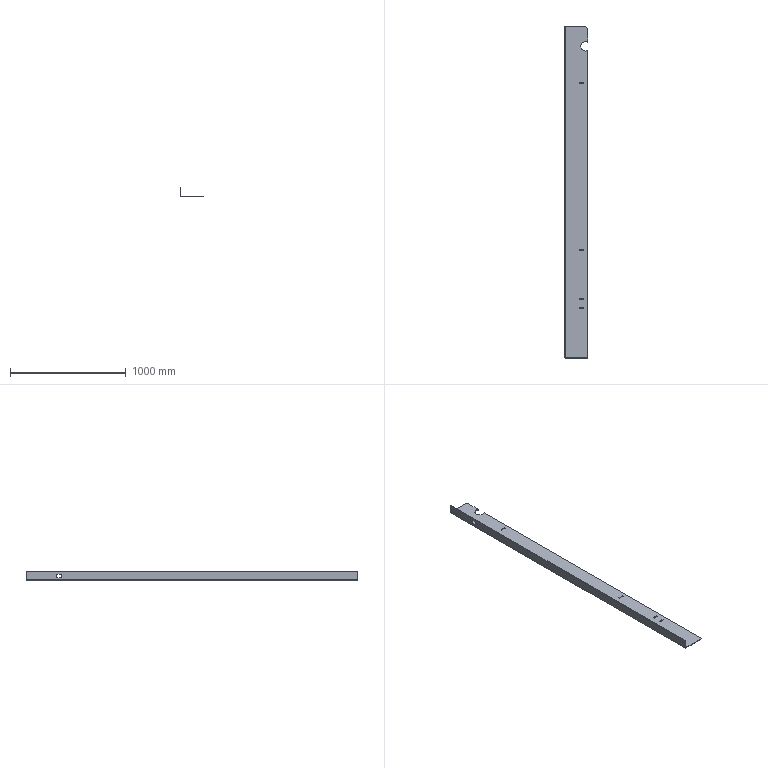Component | SolidWorks | ForkliftSidePlate,Left-1 | 1 solid | 42 faces | volume 3928487 mm3 | plane 34 | cylinder 8 | commonest cylinder face diameters 80.5 x3 30 x3 8 x1 18 x1 | material Q235